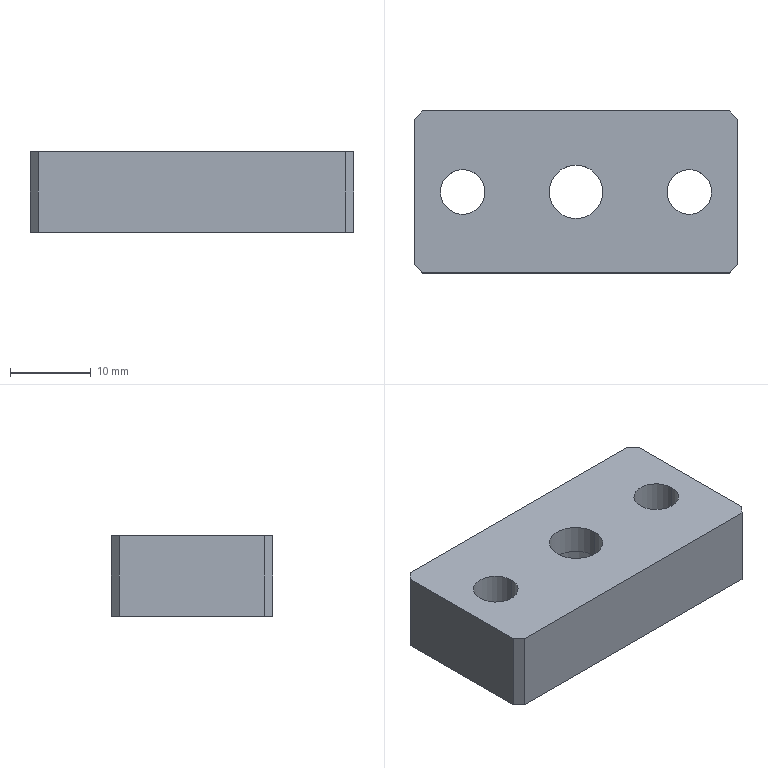Component | SolidWorks | 002MaterialPickingModuleB-1_J-004-1 | 1 solid | 25 faces | box 40 x 20 x 10 mm | volume 6182 mm3 | plane 13 | cylinder 12 | commonest cylinder face diameters 10 x4 5.5 x4 11 x2 6.6 x2 | material 45
build123d program:
from build123d import *

# Parameters (mm, degrees)
SKETCH1_W                                       = 40
SKETCH1_H                                       = 20
BOSS_EXTRUDE1_DEPTH                             = 10
M6_HEX_SOCKET_HEAD_CAP_SCREW_CBORE1_D           = 6.6
M6_HEX_SOCKET_HEAD_CAP_SCREW_CBORE1_CBORE_D     = 11
M6_HEX_SOCKET_HEAD_CAP_SCREW_CBORE1_CBORE_DEPTH = 6.4
M5_HEX_SOCKET_HEAD_CAP_SCREW_CBORE1_D           = 5.5
M5_HEX_SOCKET_HEAD_CAP_SCREW_CBORE1_CBORE_D     = 10
M5_HEX_SOCKET_HEAD_CAP_SCREW_CBORE1_CBORE_DEPTH = 5.4
CHAMFER1_SIZE                                   = 1


with BuildPart() as part:
    # Sketch1 → Boss-Extrude1 (new body)
    with BuildSketch(Plane.XY):
        Rectangle(SKETCH1_W, SKETCH1_H)
    extrude(amount=BOSS_EXTRUDE1_DEPTH)

    # M6 Hex Socket Head Cap Screw CBORE1 (through all)
    with Locations(Plane.XY.offset(10)):
        with Locations((0, 0)):
            CounterBoreHole(M6_HEX_SOCKET_HEAD_CAP_SCREW_CBORE1_D / 2, M6_HEX_SOCKET_HEAD_CAP_SCREW_CBORE1_CBORE_D / 2, M6_HEX_SOCKET_HEAD_CAP_SCREW_CBORE1_CBORE_DEPTH)

    # M5 Hex Socket Head Cap Screw CBORE1 (through all)
    with Locations(Plane.XY.offset(10)):
        with Locations((-14, 0), (14, 0)):
            CounterBoreHole(M5_HEX_SOCKET_HEAD_CAP_SCREW_CBORE1_D / 2, M5_HEX_SOCKET_HEAD_CAP_SCREW_CBORE1_CBORE_D / 2, M5_HEX_SOCKET_HEAD_CAP_SCREW_CBORE1_CBORE_DEPTH)

    # Chamfer1
    chamfer1_edges = [part.edges().sort_by_distance(p)[0] for p in [
        (-20, 10, 5),
        (20, 10, 5),
        (20, -10, 5),
        (-20, -10, 5),
    ]]
    chamfer(chamfer1_edges, length=CHAMFER1_SIZE)


solid = part.part

# Placed as in the assembly
solid = solid.moved(Location((70.325, 203.019, 113.231), (180, 0, 0)))
STEP:
#1=CARTESIAN_POINT('',(3.517,7.993,4.277));
#2=VERTEX_POINT('',#1);
#3=CARTESIAN_POINT('',(3.123,7.993,4.277));
#4=VERTEX_POINT('',#3);
#5=CARTESIAN_POINT('',(3.32,7.993,4.277));
#6=DIRECTION('',(0.,0.,-1.));
#7=DIRECTION('',(-1.,0.,0.));
#8=AXIS2_PLACEMENT_3D('',#5,#6,#7);
#9=CIRCLE('',#8,0.1969);
#10=EDGE_CURVE('',#2,#4,#9,.T.);
#11=ORIENTED_EDGE('',*,*,#10,.F.);
#12=CARTESIAN_POINT('',(3.517,7.993,4.064));
#13=VERTEX_POINT('',#12);
#14=CARTESIAN_POINT('',(3.517,7.993,4.064));
#15=DIRECTION('',(0.,0.,-1.));
#16=VECTOR('',#15,39.37);
#17=LINE('',#14,#16);
#18=EDGE_CURVE('',#2,#13,#17,.T.);
#19=ORIENTED_EDGE('',*,*,#18,.T.);
#20=CARTESIAN_POINT('',(3.123,7.993,4.064));
#21=VERTEX_POINT('',#20);
#22=CARTESIAN_POINT('',(3.32,7.993,4.064));
#23=DIRECTION('',(0.,0.,-1.));
#24=DIRECTION('',(-1.,0.,0.));
#25=AXIS2_PLACEMENT_3D('',#22,#23,#24);
#26=CIRCLE('',#25,0.1969);
#27=EDGE_CURVE('',#13,#21,#26,.T.);
#28=ORIENTED_EDGE('',*,*,#27,.T.);
#29=CARTESIAN_POINT('',(3.123,7.993,4.064));
#30=DIRECTION('',(0.,0.,-1.));
#31=VECTOR('',#30,39.37);
#32=LINE('',#29,#31);
#33=EDGE_CURVE('',#4,#21,#32,.T.);
#34=ORIENTED_EDGE('',*,*,#33,.F.);
#35=EDGE_LOOP('',(#11,#19,#28,#34));
#36=FACE_OUTER_BOUND('',#35,.T.);
#37=CARTESIAN_POINT('',(3.32,7.993,4.064));
#38=DIRECTION('',(0.,0.,-1.));
#39=DIRECTION('',(-1.,0.,0.));
#40=AXIS2_PLACEMENT_3D('',#37,#38,#39);
#41=CYLINDRICAL_SURFACE('',#40,0.1969);
#42=ADVANCED_FACE('',(#36),#41,.F.);
#43=CARTESIAN_POINT('',(3.428,7.993,4.458));
#44=VERTEX_POINT('',#43);
#45=CARTESIAN_POINT('',(3.212,7.993,4.458));
#46=VERTEX_POINT('',#45);
#47=CARTESIAN_POINT('',(3.32,7.993,4.458));
#48=DIRECTION('',(0.,0.,-1.));
#49=DIRECTION('',(-1.,0.,0.));
#50=AXIS2_PLACEMENT_3D('',#47,#48,#49);
#51=CIRCLE('',#50,0.1083);
#52=EDGE_CURVE('',#44,#46,#51,.T.);
#53=ORIENTED_EDGE('',*,*,#52,.F.);
#54=CARTESIAN_POINT('',(3.428,7.993,4.277));
#55=VERTEX_POINT('',#54);
#56=CARTESIAN_POINT('',(3.428,7.993,4.064));
#57=DIRECTION('',(0.,0.,-1.));
#58=VECTOR('',#57,39.37);
#59=LINE('',#56,#58);
#60=EDGE_CURVE('',#44,#55,#59,.T.);
#61=ORIENTED_EDGE('',*,*,#60,.T.);
#62=CARTESIAN_POINT('',(3.212,7.993,4.277));
#63=VERTEX_POINT('',#62);
#64=CARTESIAN_POINT('',(3.32,7.993,4.277));
#65=DIRECTION('',(0.,0.,-1.));
#66=DIRECTION('',(-1.,0.,0.));
#67=AXIS2_PLACEMENT_3D('',#64,#65,#66);
#68=CIRCLE('',#67,0.1083);
#69=EDGE_CURVE('',#55,#63,#68,.T.);
#70=ORIENTED_EDGE('',*,*,#69,.T.);
#71=CARTESIAN_POINT('',(3.212,7.993,4.064));
#72=DIRECTION('',(0.,0.,-1.));
#73=VECTOR('',#72,39.37);
#74=LINE('',#71,#73);
#75=EDGE_CURVE('',#46,#63,#74,.T.);
#76=ORIENTED_EDGE('',*,*,#75,.F.);
#77=EDGE_LOOP('',(#53,#61,#70,#76));
#78=FACE_OUTER_BOUND('',#77,.T.);
#79=CARTESIAN_POINT('',(3.32,7.993,4.064));
#80=DIRECTION('',(0.,0.,-1.));
#81=DIRECTION('',(-1.,0.,0.));
#82=AXIS2_PLACEMENT_3D('',#79,#80,#81);
#83=CYLINDRICAL_SURFACE('',#82,0.1083);
#84=ADVANCED_FACE('',(#78),#83,.F.);
#85=CARTESIAN_POINT('',(2.414,7.993,4.277));
#86=VERTEX_POINT('',#85);
#87=CARTESIAN_POINT('',(2.021,7.993,4.277));
#88=VERTEX_POINT('',#87);
#89=CARTESIAN_POINT('',(2.218,7.993,4.277));
#90=DIRECTION('',(0.,0.,-1.));
#91=DIRECTION('',(-1.,0.,0.));
#92=AXIS2_PLACEMENT_3D('',#89,#90,#91);
#93=CIRCLE('',#92,0.1969);
#94=EDGE_CURVE('',#86,#88,#93,.T.);
#95=ORIENTED_EDGE('',*,*,#94,.F.);
#96=CARTESIAN_POINT('',(2.414,7.993,4.064));
#97=VERTEX_POINT('',#96);
#98=CARTESIAN_POINT('',(2.414,7.993,4.064));
#99=DIRECTION('',(0.,0.,-1.));
#100=VECTOR('',#99,39.37);
#101=LINE('',#98,#100);
#102=EDGE_CURVE('',#86,#97,#101,.T.);
#103=ORIENTED_EDGE('',*,*,#102,.T.);
#104=CARTESIAN_POINT('',(2.021,7.993,4.064));
#105=VERTEX_POINT('',#104);
#106=CARTESIAN_POINT('',(2.218,7.993,4.064));
#107=DIRECTION('',(0.,0.,-1.));
#108=DIRECTION('',(-1.,0.,0.));
#109=AXIS2_PLACEMENT_3D('',#106,#107,#108);
#110=CIRCLE('',#109,0.1969);
#111=EDGE_CURVE('',#97,#105,#110,.T.);
#112=ORIENTED_EDGE('',*,*,#111,.T.);
#113=CARTESIAN_POINT('',(2.021,7.993,4.064));
#114=DIRECTION('',(0.,0.,-1.));
#115=VECTOR('',#114,39.37);
#116=LINE('',#113,#115);
#117=EDGE_CURVE('',#88,#105,#116,.T.);
#118=ORIENTED_EDGE('',*,*,#117,.F.);
#119=EDGE_LOOP('',(#95,#103,#112,#118));
#120=FACE_OUTER_BOUND('',#119,.T.);
#121=CARTESIAN_POINT('',(2.218,7.993,4.064));
#122=DIRECTION('',(0.,0.,-1.));
#123=DIRECTION('',(-1.,0.,0.));
#124=AXIS2_PLACEMENT_3D('',#121,#122,#123);
#125=CYLINDRICAL_SURFACE('',#124,0.1969);
#126=ADVANCED_FACE('',(#120),#125,.F.);
#127=CARTESIAN_POINT('',(2.326,7.993,4.458));
#128=VERTEX_POINT('',#127);
#129=CARTESIAN_POINT('',(2.109,7.993,4.458));
#130=VERTEX_POINT('',#129);
#131=CARTESIAN_POINT('',(2.218,7.993,4.458));
#132=DIRECTION('',(0.,0.,-1.));
#133=DIRECTION('',(-1.,0.,0.));
#134=AXIS2_PLACEMENT_3D('',#131,#132,#133);
#135=CIRCLE('',#134,0.1083);
#136=EDGE_CURVE('',#128,#130,#135,.T.);
#137=ORIENTED_EDGE('',*,*,#136,.F.);
#138=CARTESIAN_POINT('',(2.326,7.993,4.277));
#139=VERTEX_POINT('',#138);
#140=CARTESIAN_POINT('',(2.326,7.993,4.064));
#141=DIRECTION('',(0.,0.,-1.));
#142=VECTOR('',#141,39.37);
#143=LINE('',#140,#142);
#144=EDGE_CURVE('',#128,#139,#143,.T.);
#145=ORIENTED_EDGE('',*,*,#144,.T.);
#146=CARTESIAN_POINT('',(2.109,7.993,4.277));
#147=VERTEX_POINT('',#146);
#148=CARTESIAN_POINT('',(2.218,7.993,4.277));
#149=DIRECTION('',(0.,0.,-1.));
#150=DIRECTION('',(-1.,0.,0.));
#151=AXIS2_PLACEMENT_3D('',#148,#149,#150);
#152=CIRCLE('',#151,0.1083);
#153=EDGE_CURVE('',#139,#147,#152,.T.);
#154=ORIENTED_EDGE('',*,*,#153,.T.);
#155=CARTESIAN_POINT('',(2.109,7.993,4.064));
#156=DIRECTION('',(0.,0.,-1.));
#157=VECTOR('',#156,39.37);
#158=LINE('',#155,#157);
#159=EDGE_CURVE('',#130,#147,#158,.T.);
#160=ORIENTED_EDGE('',*,*,#159,.F.);
#161=EDGE_LOOP('',(#137,#145,#154,#160));
#162=FACE_OUTER_BOUND('',#161,.T.);
#163=CARTESIAN_POINT('',(2.218,7.993,4.064));
#164=DIRECTION('',(0.,0.,-1.));
#165=DIRECTION('',(-1.,0.,0.));
#166=AXIS2_PLACEMENT_3D('',#163,#164,#165);
#167=CYLINDRICAL_SURFACE('',#166,0.1083);
#168=ADVANCED_FACE('',(#162),#167,.F.);
#169=CARTESIAN_POINT('',(2.985,7.993,4.316));
#170=VERTEX_POINT('',#169);
#171=CARTESIAN_POINT('',(2.552,7.993,4.316));
#172=VERTEX_POINT('',#171);
#173=CARTESIAN_POINT('',(2.769,7.993,4.316));
#174=DIRECTION('',(0.,0.,-1.));
#175=DIRECTION('',(-1.,0.,0.));
#176=AXIS2_PLACEMENT_3D('',#173,#174,#175);
#177=CIRCLE('',#176,0.2165);
#178=EDGE_CURVE('',#170,#172,#177,.T.);
#179=ORIENTED_EDGE('',*,*,#178,.F.);
#180=CARTESIAN_POINT('',(2.985,7.993,4.064));
#181=VERTEX_POINT('',#180);
#182=CARTESIAN_POINT('',(2.985,7.993,4.064));
#183=DIRECTION('',(0.,0.,-1.));
#184=VECTOR('',#183,39.37);
#185=LINE('',#182,#184);
#186=EDGE_CURVE('',#170,#181,#185,.T.);
#187=ORIENTED_EDGE('',*,*,#186,.T.);
#188=CARTESIAN_POINT('',(2.552,7.993,4.064));
#189=VERTEX_POINT('',#188);
#190=CARTESIAN_POINT('',(2.769,7.993,4.064));
#191=DIRECTION('',(0.,0.,-1.));
#192=DIRECTION('',(-1.,0.,0.));
#193=AXIS2_PLACEMENT_3D('',#190,#191,#192);
#194=CIRCLE('',#193,0.2165);
#195=EDGE_CURVE('',#181,#189,#194,.T.);
#196=ORIENTED_EDGE('',*,*,#195,.T.);
#197=CARTESIAN_POINT('',(2.552,7.993,4.064));
#198=DIRECTION('',(0.,0.,-1.));
#199=VECTOR('',#198,39.37);
#200=LINE('',#197,#199);
#201=EDGE_CURVE('',#172,#189,#200,.T.);
#202=ORIENTED_EDGE('',*,*,#201,.F.);
#203=EDGE_LOOP('',(#179,#187,#196,#202));
#204=FACE_OUTER_BOUND('',#203,.T.);
#205=CARTESIAN_POINT('',(2.769,7.993,4.064));
#206=DIRECTION('',(0.,0.,-1.));
#207=DIRECTION('',(-1.,0.,0.));
#208=AXIS2_PLACEMENT_3D('',#205,#206,#207);
#209=CYLINDRICAL_SURFACE('',#208,0.2165);
#210=ADVANCED_FACE('',(#204),#209,.F.);
#211=CARTESIAN_POINT('',(2.899,7.993,4.458));
#212=VERTEX_POINT('',#211);
#213=CARTESIAN_POINT('',(2.639,7.993,4.458));
#214=VERTEX_POINT('',#213);
#215=CARTESIAN_POINT('',(2.769,7.993,4.458));
#216=DIRECTION('',(0.,0.,-1.));
#217=DIRECTION('',(-1.,0.,0.));
#218=AXIS2_PLACEMENT_3D('',#215,#216,#217);
#219=CIRCLE('',#218,0.1299);
#220=EDGE_CURVE('',#212,#214,#219,.T.);
#221=ORIENTED_EDGE('',*,*,#220,.F.);
#222=CARTESIAN_POINT('',(2.899,7.993,4.316));
#223=VERTEX_POINT('',#222);
#224=CARTESIAN_POINT('',(2.899,7.993,4.064));
#225=DIRECTION('',(0.,0.,-1.));
#226=VECTOR('',#225,39.37);
#227=LINE('',#224,#226);
#228=EDGE_CURVE('',#212,#223,#227,.T.);
#229=ORIENTED_EDGE('',*,*,#228,.T.);
#230=CARTESIAN_POINT('',(2.639,7.993,4.316));
#231=VERTEX_POINT('',#230);
#232=CARTESIAN_POINT('',(2.769,7.993,4.316));
#233=DIRECTION('',(0.,0.,-1.));
#234=DIRECTION('',(-1.,0.,0.));
#235=AXIS2_PLACEMENT_3D('',#232,#233,#234);
#236=CIRCLE('',#235,0.1299);
#237=EDGE_CURVE('',#223,#231,#236,.T.);
#238=ORIENTED_EDGE('',*,*,#237,.T.);
#239=CARTESIAN_POINT('',(2.639,7.993,4.064));
#240=DIRECTION('',(0.,0.,-1.));
#241=VECTOR('',#240,39.37);
#242=LINE('',#239,#241);
#243=EDGE_CURVE('',#214,#231,#242,.T.);
#244=ORIENTED_EDGE('',*,*,#243,.F.);
#245=EDGE_LOOP('',(#221,#229,#238,#244));
#246=FACE_OUTER_BOUND('',#245,.T.);
#247=CARTESIAN_POINT('',(2.769,7.993,4.064));
#248=DIRECTION('',(0.,0.,-1.));
#249=DIRECTION('',(-1.,0.,0.));
#250=AXIS2_PLACEMENT_3D('',#247,#248,#249);
#251=CYLINDRICAL_SURFACE('',#250,0.1299);
#252=ADVANCED_FACE('',(#246),#251,.F.);
#253=CARTESIAN_POINT('',(3.556,8.347,4.458));
#254=VERTEX_POINT('',#253);
#255=CARTESIAN_POINT('',(3.556,7.639,4.458));
#256=VERTEX_POINT('',#255);
#257=CARTESIAN_POINT('',(3.556,7.599,4.458));
#258=DIRECTION('',(0.,-1.,0.));
#259=VECTOR('',#258,39.37);
#260=LINE('',#257,#259);
#261=EDGE_CURVE('',#254,#256,#260,.T.);
#262=ORIENTED_EDGE('',*,*,#261,.T.);
#263=CARTESIAN_POINT('',(3.556,7.639,4.064));
#264=VERTEX_POINT('',#263);
#265=CARTESIAN_POINT('',(3.556,7.639,4.064));
#266=DIRECTION('',(0.,0.,-1.));
#267=VECTOR('',#266,39.37);
#268=LINE('',#265,#267);
#269=EDGE_CURVE('',#256,#264,#268,.T.);
#270=ORIENTED_EDGE('',*,*,#269,.T.);
#271=CARTESIAN_POINT('',(3.556,8.347,4.064));
#272=VERTEX_POINT('',#271);
#273=CARTESIAN_POINT('',(3.556,7.599,4.064));
#274=DIRECTION('',(0.,-1.,0.));
#275=VECTOR('',#274,39.37);
#276=LINE('',#273,#275);
#277=EDGE_CURVE('',#272,#264,#276,.T.);
#278=ORIENTED_EDGE('',*,*,#277,.F.);
#279=CARTESIAN_POINT('',(3.556,8.347,4.064));
#280=DIRECTION('',(0.,0.,1.));
#281=VECTOR('',#280,39.37);
#282=LINE('',#279,#281);
#283=EDGE_CURVE('',#272,#254,#282,.T.);
#284=ORIENTED_EDGE('',*,*,#283,.T.);
#285=EDGE_LOOP('',(#262,#270,#278,#284));
#286=FACE_OUTER_BOUND('',#285,.T.);
#287=CARTESIAN_POINT('',(3.556,7.599,4.064));
#288=DIRECTION('',(-1.,-0.,0.));
#289=DIRECTION('',(0.,0.,1.));
#290=AXIS2_PLACEMENT_3D('',#287,#288,#289);
#291=PLANE('',#290);
#292=ADVANCED_FACE('',(#286),#291,.F.);
#293=CARTESIAN_POINT('',(3.517,7.599,4.064));
#294=VERTEX_POINT('',#293);
#295=CARTESIAN_POINT('',(2.021,7.599,4.064));
#296=VERTEX_POINT('',#295);
#297=CARTESIAN_POINT('',(1.981,7.599,4.064));
#298=DIRECTION('',(-1.,-0.,0.));
#299=VECTOR('',#298,39.37);
#300=LINE('',#297,#299);
#301=EDGE_CURVE('',#294,#296,#300,.T.);
#302=ORIENTED_EDGE('',*,*,#301,.F.);
#303=CARTESIAN_POINT('',(3.517,7.599,4.458));
#304=VERTEX_POINT('',#303);
#305=CARTESIAN_POINT('',(3.517,7.599,4.064));
#306=DIRECTION('',(0.,0.,1.));
#307=VECTOR('',#306,39.37);
#308=LINE('',#305,#307);
#309=EDGE_CURVE('',#294,#304,#308,.T.);
#310=ORIENTED_EDGE('',*,*,#309,.T.);
#311=CARTESIAN_POINT('',(2.021,7.599,4.458));
#312=VERTEX_POINT('',#311);
#313=CARTESIAN_POINT('',(1.981,7.599,4.458));
#314=DIRECTION('',(-1.,-0.,0.));
#315=VECTOR('',#314,39.37);
#316=LINE('',#313,#315);
#317=EDGE_CURVE('',#304,#312,#316,.T.);
#318=ORIENTED_EDGE('',*,*,#317,.T.);
#319=CARTESIAN_POINT('',(2.021,7.599,4.064));
#320=DIRECTION('',(0.,0.,-1.));
#321=VECTOR('',#320,39.37);
#322=LINE('',#319,#321);
#323=EDGE_CURVE('',#312,#296,#322,.T.);
#324=ORIENTED_EDGE('',*,*,#323,.T.);
#325=EDGE_LOOP('',(#302,#310,#318,#324));
#326=FACE_OUTER_BOUND('',#325,.T.);
#327=CARTESIAN_POINT('',(1.981,7.599,4.064));
#328=DIRECTION('',(-0.,1.,0.));
#329=DIRECTION('',(1.,0.,0.));
#330=AXIS2_PLACEMENT_3D('',#327,#328,#329);
#331=PLANE('',#330);
#332=ADVANCED_FACE('',(#326),#331,.F.);
#333=CARTESIAN_POINT('',(1.981,7.639,4.064));
#334=VERTEX_POINT('',#333);
#335=CARTESIAN_POINT('',(1.981,8.347,4.064));
#336=VERTEX_POINT('',#335);
#337=CARTESIAN_POINT('',(1.981,7.599,4.064));
#338=DIRECTION('',(-0.,1.,0.));
#339=VECTOR('',#338,39.37);
#340=LINE('',#337,#339);
#341=EDGE_CURVE('',#334,#336,#340,.T.);
#342=ORIENTED_EDGE('',*,*,#341,.F.);
#343=CARTESIAN_POINT('',(1.981,7.639,4.458));
#344=VERTEX_POINT('',#343);
#345=CARTESIAN_POINT('',(1.981,7.639,4.064));
#346=DIRECTION('',(0.,0.,1.));
#347=VECTOR('',#346,39.37);
#348=LINE('',#345,#347);
#349=EDGE_CURVE('',#334,#344,#348,.T.);
#350=ORIENTED_EDGE('',*,*,#349,.T.);
#351=CARTESIAN_POINT('',(1.981,8.347,4.458));
#352=VERTEX_POINT('',#351);
#353=CARTESIAN_POINT('',(1.981,7.599,4.458));
#354=DIRECTION('',(-0.,1.,0.));
#355=VECTOR('',#354,39.37);
#356=LINE('',#353,#355);
#357=EDGE_CURVE('',#344,#352,#356,.T.);
#358=ORIENTED_EDGE('',*,*,#357,.T.);
#359=CARTESIAN_POINT('',(1.981,8.347,4.064));
#360=DIRECTION('',(0.,0.,-1.));
#361=VECTOR('',#360,39.37);
#362=LINE('',#359,#361);
#363=EDGE_CURVE('',#352,#336,#362,.T.);
#364=ORIENTED_EDGE('',*,*,#363,.T.);
#365=EDGE_LOOP('',(#342,#350,#358,#364));
#366=FACE_OUTER_BOUND('',#365,.T.);
#367=CARTESIAN_POINT('',(1.981,7.599,4.064));
#368=DIRECTION('',(1.,0.,0.));
#369=DIRECTION('',(0.,0.,-1.));
#370=AXIS2_PLACEMENT_3D('',#367,#368,#369);
#371=PLANE('',#370);
#372=ADVANCED_FACE('',(#366),#371,.F.);
#373=CARTESIAN_POINT('',(2.021,8.387,4.064));
#374=VERTEX_POINT('',#373);
#375=CARTESIAN_POINT('',(3.517,8.387,4.064));
#376=VERTEX_POINT('',#375);
#377=CARTESIAN_POINT('',(1.981,8.387,4.064));
#378=DIRECTION('',(1.,0.,0.));
#379=VECTOR('',#378,39.37);
#380=LINE('',#377,#379);
#381=EDGE_CURVE('',#374,#376,#380,.T.);
#382=ORIENTED_EDGE('',*,*,#381,.F.);
#383=CARTESIAN_POINT('',(2.021,8.387,4.458));
#384=VERTEX_POINT('',#383);
#385=CARTESIAN_POINT('',(2.021,8.387,4.064));
#386=DIRECTION('',(0.,0.,1.));
#387=VECTOR('',#386,39.37);
#388=LINE('',#385,#387);
#389=EDGE_CURVE('',#374,#384,#388,.T.);
#390=ORIENTED_EDGE('',*,*,#389,.T.);
#391=CARTESIAN_POINT('',(3.517,8.387,4.458));
#392=VERTEX_POINT('',#391);
#393=CARTESIAN_POINT('',(1.981,8.387,4.458));
#394=DIRECTION('',(1.,0.,0.));
#395=VECTOR('',#394,39.37);
#396=LINE('',#393,#395);
#397=EDGE_CURVE('',#384,#392,#396,.T.);
#398=ORIENTED_EDGE('',*,*,#397,.T.);
#399=CARTESIAN_POINT('',(3.517,8.387,4.064));
#400=DIRECTION('',(0.,0.,-1.));
#401=VECTOR('',#400,39.37);
#402=LINE('',#399,#401);
#403=EDGE_CURVE('',#392,#376,#402,.T.);
#404=ORIENTED_EDGE('',*,*,#403,.T.);
#405=EDGE_LOOP('',(#382,#390,#398,#404));
#406=FACE_OUTER_BOUND('',#405,.T.);
#407=CARTESIAN_POINT('',(1.981,8.387,4.064));
#408=DIRECTION('',(0.,-1.,0.));
#409=DIRECTION('',(-1.,-0.,0.));
#410=AXIS2_PLACEMENT_3D('',#407,#408,#409);
#411=PLANE('',#410);
#412=ADVANCED_FACE('',(#406),#411,.F.);
#413=CARTESIAN_POINT('',(3.32,7.993,4.064));
#414=DIRECTION('',(0.,0.,-1.));
#415=DIRECTION('',(-1.,0.,0.));
#416=AXIS2_PLACEMENT_3D('',#413,#414,#415);
#417=CIRCLE('',#416,0.1969);
#418=EDGE_CURVE('',#21,#13,#417,.T.);
#419=ORIENTED_EDGE('',*,*,#418,.F.);
#420=ORIENTED_EDGE('',*,*,#27,.F.);
#421=EDGE_LOOP('',(#419,#420));
#422=FACE_BOUND('',#421,.T.);
#423=CARTESIAN_POINT('',(2.218,7.993,4.064));
#424=DIRECTION('',(0.,0.,-1.));
#425=DIRECTION('',(-1.,0.,0.));
#426=AXIS2_PLACEMENT_3D('',#423,#424,#425);
#427=CIRCLE('',#426,0.1969);
#428=EDGE_CURVE('',#105,#97,#427,.T.);
#429=ORIENTED_EDGE('',*,*,#428,.F.);
#430=ORIENTED_EDGE('',*,*,#111,.F.);
#431=EDGE_LOOP('',(#429,#430));
#432=FACE_BOUND('',#431,.T.);
#433=CARTESIAN_POINT('',(2.769,7.993,4.064));
#434=DIRECTION('',(0.,0.,-1.));
#435=DIRECTION('',(-1.,0.,0.));
#436=AXIS2_PLACEMENT_3D('',#433,#434,#435);
#437=CIRCLE('',#436,0.2165);
#438=EDGE_CURVE('',#189,#181,#437,.T.);
#439=ORIENTED_EDGE('',*,*,#438,.F.);
#440=ORIENTED_EDGE('',*,*,#195,.F.);
#441=EDGE_LOOP('',(#439,#440));
#442=FACE_BOUND('',#441,.T.);
#443=ORIENTED_EDGE('',*,*,#277,.T.);
#444=CARTESIAN_POINT('',(3.34,7.422,4.064));
#445=DIRECTION('',(-0.7071,-0.7071,0.));
#446=VECTOR('',#445,39.37);
#447=LINE('',#444,#446);
#448=EDGE_CURVE('',#264,#294,#447,.T.);
#449=ORIENTED_EDGE('',*,*,#448,.T.);
#450=ORIENTED_EDGE('',*,*,#301,.T.);
#451=CARTESIAN_POINT('',(2.198,7.422,4.064));
#452=DIRECTION('',(-0.7071,0.7071,0.));
#453=VECTOR('',#452,39.37);
#454=LINE('',#451,#453);
#455=EDGE_CURVE('',#296,#334,#454,.T.);
#456=ORIENTED_EDGE('',*,*,#455,.T.);
#457=ORIENTED_EDGE('',*,*,#341,.T.);
#458=CARTESIAN_POINT('',(2.198,8.564,4.064));
#459=DIRECTION('',(0.7071,0.7071,0.));
#460=VECTOR('',#459,39.37);
#461=LINE('',#458,#460);
#462=EDGE_CURVE('',#336,#374,#461,.T.);
#463=ORIENTED_EDGE('',*,*,#462,.T.);
#464=ORIENTED_EDGE('',*,*,#381,.T.);
#465=CARTESIAN_POINT('',(3.34,8.564,4.064));
#466=DIRECTION('',(0.7071,-0.7071,0.));
#467=VECTOR('',#466,39.37);
#468=LINE('',#465,#467);
#469=EDGE_CURVE('',#376,#272,#468,.T.);
#470=ORIENTED_EDGE('',*,*,#469,.T.);
#471=EDGE_LOOP('',(#443,#449,#450,#456,#457,#463,#464,#470));
#472=FACE_OUTER_BOUND('',#471,.T.);
#473=CARTESIAN_POINT('',(2.769,7.993,4.064));
#474=DIRECTION('',(0.,0.,-1.));
#475=DIRECTION('',(-1.,-0.,0.));
#476=AXIS2_PLACEMENT_3D('',#473,#474,#475);
#477=PLANE('',#476);
#478=ADVANCED_FACE('',(#422,#432,#442,#472),#477,.T.);
#479=CARTESIAN_POINT('',(3.32,7.993,4.458));
#480=DIRECTION('',(0.,0.,-1.));
#481=DIRECTION('',(-1.,0.,0.));
#482=AXIS2_PLACEMENT_3D('',#479,#480,#481);
#483=CIRCLE('',#482,0.1083);
#484=EDGE_CURVE('',#46,#44,#483,.T.);
#485=ORIENTED_EDGE('',*,*,#484,.T.);
#486=ORIENTED_EDGE('',*,*,#52,.T.);
#487=EDGE_LOOP('',(#485,#486));
#488=FACE_BOUND('',#487,.T.);
#489=CARTESIAN_POINT('',(2.218,7.993,4.458));
#490=DIRECTION('',(0.,0.,-1.));
#491=DIRECTION('',(-1.,0.,0.));
#492=AXIS2_PLACEMENT_3D('',#489,#490,#491);
#493=CIRCLE('',#492,0.1083);
#494=EDGE_CURVE('',#130,#128,#493,.T.);
#495=ORIENTED_EDGE('',*,*,#494,.T.);
#496=ORIENTED_EDGE('',*,*,#136,.T.);
#497=EDGE_LOOP('',(#495,#496));
#498=FACE_BOUND('',#497,.T.);
#499=CARTESIAN_POINT('',(2.769,7.993,4.458));
#500=DIRECTION('',(0.,0.,-1.));
#501=DIRECTION('',(-1.,0.,0.));
#502=AXIS2_PLACEMENT_3D('',#499,#500,#501);
#503=CIRCLE('',#502,0.1299);
#504=EDGE_CURVE('',#214,#212,#503,.T.);
#505=ORIENTED_EDGE('',*,*,#504,.T.);
#506=ORIENTED_EDGE('',*,*,#220,.T.);
#507=EDGE_LOOP('',(#505,#506));
#508=FACE_BOUND('',#507,.T.);
#509=ORIENTED_EDGE('',*,*,#317,.F.);
#510=CARTESIAN_POINT('',(3.517,7.599,4.458));
#511=DIRECTION('',(0.7071,0.7071,0.));
#512=VECTOR('',#511,39.37);
#513=LINE('',#510,#512);
#514=EDGE_CURVE('',#304,#256,#513,.T.);
#515=ORIENTED_EDGE('',*,*,#514,.T.);
#516=ORIENTED_EDGE('',*,*,#261,.F.);
#517=CARTESIAN_POINT('',(3.556,8.347,4.458));
#518=DIRECTION('',(-0.7071,0.7071,0.));
#519=VECTOR('',#518,39.37);
#520=LINE('',#517,#519);
#521=EDGE_CURVE('',#254,#392,#520,.T.);
#522=ORIENTED_EDGE('',*,*,#521,.T.);
#523=ORIENTED_EDGE('',*,*,#397,.F.);
#524=CARTESIAN_POINT('',(2.021,8.387,4.458));
#525=DIRECTION('',(-0.7071,-0.7071,0.));
#526=VECTOR('',#525,39.37);
#527=LINE('',#524,#526);
#528=EDGE_CURVE('',#384,#352,#527,.T.);
#529=ORIENTED_EDGE('',*,*,#528,.T.);
#530=ORIENTED_EDGE('',*,*,#357,.F.);
#531=CARTESIAN_POINT('',(1.981,7.639,4.458));
#532=DIRECTION('',(0.7071,-0.7071,0.));
#533=VECTOR('',#532,39.37);
#534=LINE('',#531,#533);
#535=EDGE_CURVE('',#344,#312,#534,.T.);
#536=ORIENTED_EDGE('',*,*,#535,.T.);
#537=EDGE_LOOP('',(#509,#515,#516,#522,#523,#529,#530,#536));
#538=FACE_OUTER_BOUND('',#537,.T.);
#539=CARTESIAN_POINT('',(2.769,7.993,4.458));
#540=DIRECTION('',(0.,0.,-1.));
#541=DIRECTION('',(-1.,-0.,0.));
#542=AXIS2_PLACEMENT_3D('',#539,#540,#541);
#543=PLANE('',#542);
#544=ADVANCED_FACE('',(#488,#498,#508,#538),#543,.F.);
#545=ORIENTED_EDGE('',*,*,#228,.F.);
#546=ORIENTED_EDGE('',*,*,#504,.F.);
#547=ORIENTED_EDGE('',*,*,#243,.T.);
#548=CARTESIAN_POINT('',(2.769,7.993,4.316));
#549=DIRECTION('',(0.,0.,-1.));
#550=DIRECTION('',(-1.,0.,0.));
#551=AXIS2_PLACEMENT_3D('',#548,#549,#550);
#552=CIRCLE('',#551,0.1299);
#553=EDGE_CURVE('',#231,#223,#552,.T.);
#554=ORIENTED_EDGE('',*,*,#553,.T.);
#555=EDGE_LOOP('',(#545,#546,#547,#554));
#556=FACE_OUTER_BOUND('',#555,.T.);
#557=CARTESIAN_POINT('',(2.769,7.993,4.064));
#558=DIRECTION('',(0.,0.,-1.));
#559=DIRECTION('',(-1.,0.,0.));
#560=AXIS2_PLACEMENT_3D('',#557,#558,#559);
#561=CYLINDRICAL_SURFACE('',#560,0.1299);
#562=ADVANCED_FACE('',(#556),#561,.F.);
#563=ORIENTED_EDGE('',*,*,#553,.F.);
#564=ORIENTED_EDGE('',*,*,#237,.F.);
#565=EDGE_LOOP('',(#563,#564));
#566=FACE_BOUND('',#565,.T.);
#567=CARTESIAN_POINT('',(2.769,7.993,4.316));
#568=DIRECTION('',(0.,0.,-1.));
#569=DIRECTION('',(-1.,0.,0.));
#570=AXIS2_PLACEMENT_3D('',#567,#568,#569);
#571=CIRCLE('',#570,0.2165);
#572=EDGE_CURVE('',#172,#170,#571,.T.);
#573=ORIENTED_EDGE('',*,*,#572,.T.);
#574=ORIENTED_EDGE('',*,*,#178,.T.);
#575=EDGE_LOOP('',(#573,#574));
#576=FACE_OUTER_BOUND('',#575,.T.);
#577=CARTESIAN_POINT('',(2.639,7.993,4.316));
#578=DIRECTION('',(0.,0.,1.));
#579=DIRECTION('',(1.,0.,0.));
#580=AXIS2_PLACEMENT_3D('',#577,#578,#579);
#581=PLANE('',#580);
#582=ADVANCED_FACE('',(#566,#576),#581,.F.);
#583=ORIENTED_EDGE('',*,*,#186,.F.);
#584=ORIENTED_EDGE('',*,*,#572,.F.);
#585=ORIENTED_EDGE('',*,*,#201,.T.);
#586=ORIENTED_EDGE('',*,*,#438,.T.);
#587=EDGE_LOOP('',(#583,#584,#585,#586));
#588=FACE_OUTER_BOUND('',#587,.T.);
#589=CARTESIAN_POINT('',(2.769,7.993,4.064));
#590=DIRECTION('',(0.,0.,-1.));
#591=DIRECTION('',(-1.,0.,0.));
#592=AXIS2_PLACEMENT_3D('',#589,#590,#591);
#593=CYLINDRICAL_SURFACE('',#592,0.2165);
#594=ADVANCED_FACE('',(#588),#593,.F.);
#595=ORIENTED_EDGE('',*,*,#144,.F.);
#596=ORIENTED_EDGE('',*,*,#494,.F.);
#597=ORIENTED_EDGE('',*,*,#159,.T.);
#598=CARTESIAN_POINT('',(2.218,7.993,4.277));
#599=DIRECTION('',(0.,0.,-1.));
#600=DIRECTION('',(-1.,0.,0.));
#601=AXIS2_PLACEMENT_3D('',#598,#599,#600);
#602=CIRCLE('',#601,0.1083);
#603=EDGE_CURVE('',#147,#139,#602,.T.);
#604=ORIENTED_EDGE('',*,*,#603,.T.);
#605=EDGE_LOOP('',(#595,#596,#597,#604));
#606=FACE_OUTER_BOUND('',#605,.T.);
#607=CARTESIAN_POINT('',(2.218,7.993,4.064));
#608=DIRECTION('',(0.,0.,-1.));
#609=DIRECTION('',(-1.,0.,0.));
#610=AXIS2_PLACEMENT_3D('',#607,#608,#609);
#611=CYLINDRICAL_SURFACE('',#610,0.1083);
#612=ADVANCED_FACE('',(#606),#611,.F.);
#613=ORIENTED_EDGE('',*,*,#603,.F.);
#614=ORIENTED_EDGE('',*,*,#153,.F.);
#615=EDGE_LOOP('',(#613,#614));
#616=FACE_BOUND('',#615,.T.);
#617=CARTESIAN_POINT('',(2.218,7.993,4.277));
#618=DIRECTION('',(0.,0.,-1.));
#619=DIRECTION('',(-1.,0.,0.));
#620=AXIS2_PLACEMENT_3D('',#617,#618,#619);
#621=CIRCLE('',#620,0.1969);
#622=EDGE_CURVE('',#88,#86,#621,.T.);
#623=ORIENTED_EDGE('',*,*,#622,.T.);
#624=ORIENTED_EDGE('',*,*,#94,.T.);
#625=EDGE_LOOP('',(#623,#624));
#626=FACE_OUTER_BOUND('',#625,.T.);
#627=CARTESIAN_POINT('',(2.109,7.993,4.277));
#628=DIRECTION('',(0.,0.,1.));
#629=DIRECTION('',(1.,0.,0.));
#630=AXIS2_PLACEMENT_3D('',#627,#628,#629);
#631=PLANE('',#630);
#632=ADVANCED_FACE('',(#616,#626),#631,.F.);
#633=ORIENTED_EDGE('',*,*,#102,.F.);
#634=ORIENTED_EDGE('',*,*,#622,.F.);
#635=ORIENTED_EDGE('',*,*,#117,.T.);
#636=ORIENTED_EDGE('',*,*,#428,.T.);
#637=EDGE_LOOP('',(#633,#634,#635,#636));
#638=FACE_OUTER_BOUND('',#637,.T.);
#639=CARTESIAN_POINT('',(2.218,7.993,4.064));
#640=DIRECTION('',(0.,0.,-1.));
#641=DIRECTION('',(-1.,0.,0.));
#642=AXIS2_PLACEMENT_3D('',#639,#640,#641);
#643=CYLINDRICAL_SURFACE('',#642,0.1969);
#644=ADVANCED_FACE('',(#638),#643,.F.);
#645=ORIENTED_EDGE('',*,*,#60,.F.);
#646=ORIENTED_EDGE('',*,*,#484,.F.);
#647=ORIENTED_EDGE('',*,*,#75,.T.);
#648=CARTESIAN_POINT('',(3.32,7.993,4.277));
#649=DIRECTION('',(0.,0.,-1.));
#650=DIRECTION('',(-1.,0.,0.));
#651=AXIS2_PLACEMENT_3D('',#648,#649,#650);
#652=CIRCLE('',#651,0.1083);
#653=EDGE_CURVE('',#63,#55,#652,.T.);
#654=ORIENTED_EDGE('',*,*,#653,.T.);
#655=EDGE_LOOP('',(#645,#646,#647,#654));
#656=FACE_OUTER_BOUND('',#655,.T.);
#657=CARTESIAN_POINT('',(3.32,7.993,4.064));
#658=DIRECTION('',(0.,0.,-1.));
#659=DIRECTION('',(-1.,0.,0.));
#660=AXIS2_PLACEMENT_3D('',#657,#658,#659);
#661=CYLINDRICAL_SURFACE('',#660,0.1083);
#662=ADVANCED_FACE('',(#656),#661,.F.);
#663=ORIENTED_EDGE('',*,*,#653,.F.);
#664=ORIENTED_EDGE('',*,*,#69,.F.);
#665=EDGE_LOOP('',(#663,#664));
#666=FACE_BOUND('',#665,.T.);
#667=CARTESIAN_POINT('',(3.32,7.993,4.277));
#668=DIRECTION('',(0.,0.,-1.));
#669=DIRECTION('',(-1.,0.,0.));
#670=AXIS2_PLACEMENT_3D('',#667,#668,#669);
#671=CIRCLE('',#670,0.1969);
#672=EDGE_CURVE('',#4,#2,#671,.T.);
#673=ORIENTED_EDGE('',*,*,#672,.T.);
#674=ORIENTED_EDGE('',*,*,#10,.T.);
#675=EDGE_LOOP('',(#673,#674));
#676=FACE_OUTER_BOUND('',#675,.T.);
#677=CARTESIAN_POINT('',(3.212,7.993,4.277));
#678=DIRECTION('',(0.,0.,1.));
#679=DIRECTION('',(1.,0.,0.));
#680=AXIS2_PLACEMENT_3D('',#677,#678,#679);
#681=PLANE('',#680);
#682=ADVANCED_FACE('',(#666,#676),#681,.F.);
#683=ORIENTED_EDGE('',*,*,#18,.F.);
#684=ORIENTED_EDGE('',*,*,#672,.F.);
#685=ORIENTED_EDGE('',*,*,#33,.T.);
#686=ORIENTED_EDGE('',*,*,#418,.T.);
#687=EDGE_LOOP('',(#683,#684,#685,#686));
#688=FACE_OUTER_BOUND('',#687,.T.);
#689=CARTESIAN_POINT('',(3.32,7.993,4.064));
#690=DIRECTION('',(0.,0.,-1.));
#691=DIRECTION('',(-1.,0.,0.));
#692=AXIS2_PLACEMENT_3D('',#689,#690,#691);
#693=CYLINDRICAL_SURFACE('',#692,0.1969);
#694=ADVANCED_FACE('',(#688),#693,.F.);
#695=ORIENTED_EDGE('',*,*,#448,.F.);
#696=ORIENTED_EDGE('',*,*,#269,.F.);
#697=ORIENTED_EDGE('',*,*,#514,.F.);
#698=ORIENTED_EDGE('',*,*,#309,.F.);
#699=EDGE_LOOP('',(#695,#696,#697,#698));
#700=FACE_OUTER_BOUND('',#699,.T.);
#701=CARTESIAN_POINT('',(3.517,7.599,4.064));
#702=DIRECTION('',(-0.7071,0.7071,0.));
#703=DIRECTION('',(0.,0.,1.));
#704=AXIS2_PLACEMENT_3D('',#701,#702,#703);
#705=PLANE('',#704);
#706=ADVANCED_FACE('',(#700),#705,.F.);
#707=ORIENTED_EDGE('',*,*,#455,.F.);
#708=ORIENTED_EDGE('',*,*,#323,.F.);
#709=ORIENTED_EDGE('',*,*,#535,.F.);
#710=ORIENTED_EDGE('',*,*,#349,.F.);
#711=EDGE_LOOP('',(#707,#708,#709,#710));
#712=FACE_OUTER_BOUND('',#711,.T.);
#713=CARTESIAN_POINT('',(1.981,7.639,4.064));
#714=DIRECTION('',(0.7071,0.7071,0.));
#715=DIRECTION('',(0.,0.,1.));
#716=AXIS2_PLACEMENT_3D('',#713,#714,#715);
#717=PLANE('',#716);
#718=ADVANCED_FACE('',(#712),#717,.F.);
#719=ORIENTED_EDGE('',*,*,#462,.F.);
#720=ORIENTED_EDGE('',*,*,#363,.F.);
#721=ORIENTED_EDGE('',*,*,#528,.F.);
#722=ORIENTED_EDGE('',*,*,#389,.F.);
#723=EDGE_LOOP('',(#719,#720,#721,#722));
#724=FACE_OUTER_BOUND('',#723,.T.);
#725=CARTESIAN_POINT('',(2.021,8.387,4.064));
#726=DIRECTION('',(0.7071,-0.7071,0.));
#727=DIRECTION('',(0.,0.,1.));
#728=AXIS2_PLACEMENT_3D('',#725,#726,#727);
#729=PLANE('',#728);
#730=ADVANCED_FACE('',(#724),#729,.F.);
#731=ORIENTED_EDGE('',*,*,#469,.F.);
#732=ORIENTED_EDGE('',*,*,#403,.F.);
#733=ORIENTED_EDGE('',*,*,#521,.F.);
#734=ORIENTED_EDGE('',*,*,#283,.F.);
#735=EDGE_LOOP('',(#731,#732,#733,#734));
#736=FACE_OUTER_BOUND('',#735,.T.);
#737=CARTESIAN_POINT('',(3.556,8.347,4.064));
#738=DIRECTION('',(-0.7071,-0.7071,0.));
#739=DIRECTION('',(0.,0.,1.));
#740=AXIS2_PLACEMENT_3D('',#737,#738,#739);
#741=PLANE('',#740);
#742=ADVANCED_FACE('',(#736),#741,.F.);
#743=CLOSED_SHELL('',(#42,#84,#126,#168,#210,#252,#292,#332,#372,#412,#478,#544,#562,#582,#594,#612,#632,#644,#662,#682,#694,#706,#718,#730,#742));
#744=MANIFOLD_SOLID_BREP('',#743);
#745=CARTESIAN_POINT('',(0.,0.,0.));
#746=DIRECTION('',(0.,0.,1.));
#747=DIRECTION('',(1.,0.,0.));
#748=AXIS2_PLACEMENT_3D('',#745,#746,#747);
#749=(LENGTH_UNIT()NAMED_UNIT(*)SI_UNIT($,.METRE.));
#750=LENGTH_MEASURE_WITH_UNIT(LENGTH_MEASURE(0.0254),#749);
#751=DIMENSIONAL_EXPONENTS(1.,0.,0.,0.,0.,0.,0.);
#752=(CONVERSION_BASED_UNIT('',#750)LENGTH_UNIT()NAMED_UNIT(#751));
#753=UNCERTAINTY_MEASURE_WITH_UNIT(LENGTH_MEASURE(0.00001),#752,'','');
#754=(NAMED_UNIT(*)PLANE_ANGLE_UNIT()SI_UNIT($,.RADIAN.));
#755=(NAMED_UNIT(*)SI_UNIT($,.STERADIAN.)SOLID_ANGLE_UNIT());
#756=(GEOMETRIC_REPRESENTATION_CONTEXT(3)GLOBAL_UNCERTAINTY_ASSIGNED_CONTEXT((#753))GLOBAL_UNIT_ASSIGNED_CONTEXT((#752,#754,#755))REPRESENTATION_CONTEXT('',''));
#757=ADVANCED_BREP_SHAPE_REPRESENTATION('',(#744,#748),#756);
#758=COLOUR_RGB('',0.7922,0.8196,0.9333);
#759=FILL_AREA_STYLE_COLOUR('',#758);
#760=FILL_AREA_STYLE('',(#759));
#761=SURFACE_STYLE_FILL_AREA(#760);
#762=SURFACE_SIDE_STYLE('',(#761));
#763=SURFACE_STYLE_USAGE(.BOTH.,#762);
#764=PRESENTATION_STYLE_ASSIGNMENT((#763));
#765=STYLED_ITEM('',(#764),#744);
#766=PRESENTATION_LAYER_ASSIGNMENT('','',(#765));
#767=(LENGTH_UNIT()NAMED_UNIT(*)SI_UNIT($,.METRE.));
#768=LENGTH_MEASURE_WITH_UNIT(LENGTH_MEASURE(0.0254),#767);
#769=DIMENSIONAL_EXPONENTS(1.,0.,0.,0.,0.,0.,0.);
#770=(CONVERSION_BASED_UNIT('',#768)LENGTH_UNIT()NAMED_UNIT(#769));
#771=UNCERTAINTY_MEASURE_WITH_UNIT(LENGTH_MEASURE(0.00001),#770,'','');
#772=(NAMED_UNIT(*)PLANE_ANGLE_UNIT()SI_UNIT($,.RADIAN.));
#773=(NAMED_UNIT(*)SI_UNIT($,.STERADIAN.)SOLID_ANGLE_UNIT());
#774=(GEOMETRIC_REPRESENTATION_CONTEXT(3)GLOBAL_UNCERTAINTY_ASSIGNED_CONTEXT((#771))GLOBAL_UNIT_ASSIGNED_CONTEXT((#770,#772,#773))REPRESENTATION_CONTEXT('',''));
#775=MECHANICAL_DESIGN_GEOMETRIC_PRESENTATION_REPRESENTATION('',(#765),#774);